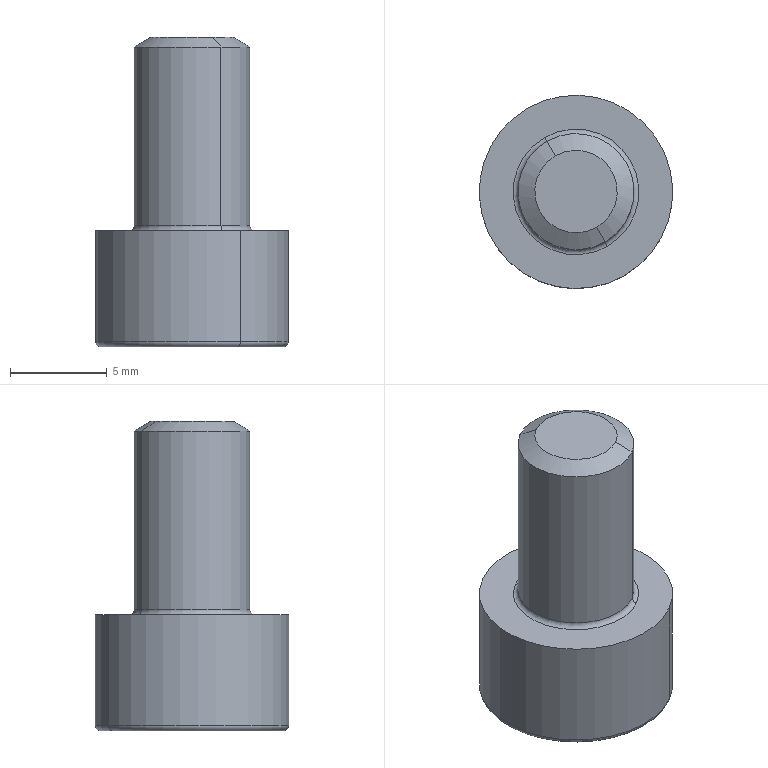Component | NX | HEX_SOCKET_SCREW_M6X10_4 | 1 solid | 20 faces | volume 686 mm3 | plane 10 | torus 4 | cylinder 4 | cone 2 | commonest cylinder face diameters 10 x2 6 x2